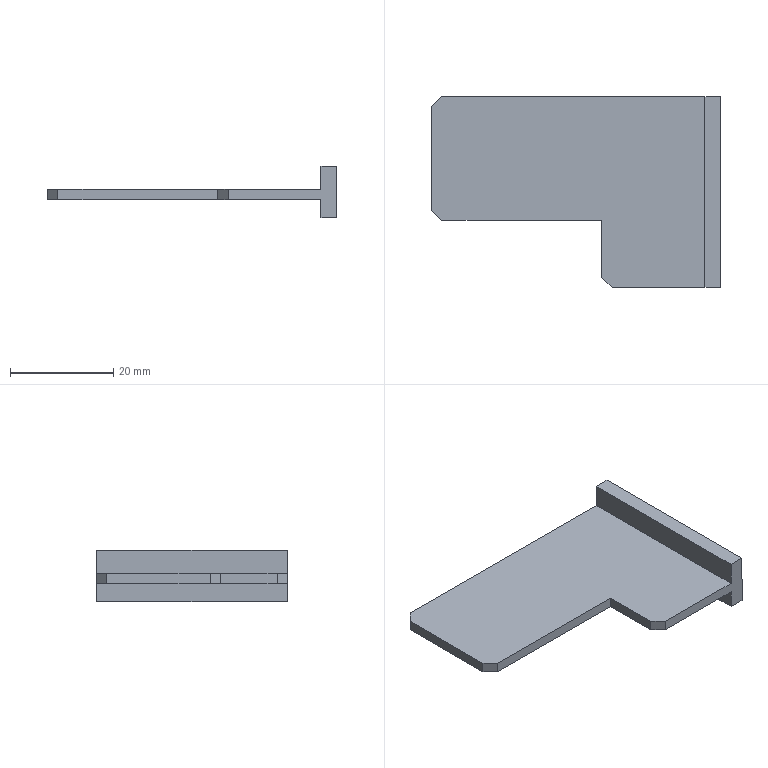Component | SolidWorks | 2023-12-12-28-1 | 1 solid | 15 faces | box 56 x 37 x 10 mm | volume 4162 mm3 | plane 15
build123d program:
from build123d import *

# Parameters (mm, degrees)
SKETCH1_W           = 37
SKETCH1_H           = 56
BOSS_EXTRUDE1_DEPTH = 10
SKETCH2_W           = 4.5
SKETCH2_H           = 53
SKETCH2_W_2         = 3.5
CUT_EXTRUDE1_DEPTH  = 68.86
SKETCH3_W           = 13
SKETCH3_H           = 33
CUT_EXTRUDE2_DEPTH  = 10
CHAMFER1_SIZE       = 2


with BuildPart() as part:
    # Sketch1 → Boss-Extrude1 (new body)
    with BuildSketch(Plane.XY):
        with Locations((18.5, 28)):
            Rectangle(SKETCH1_W, SKETCH1_H)
    extrude(amount=BOSS_EXTRUDE1_DEPTH)

    # Sketch2 → Cut-Extrude1 (cut, through all)
    with BuildSketch(Plane(origin=(37, 0, 0), x_dir=(0, 0, -1), z_dir=(1, 0, 0))):
        with Locations((-7.75, 29.5)):
            Rectangle(SKETCH2_W, SKETCH2_H)
        with Locations((-1.75, 29.5)):
            Rectangle(SKETCH2_W_2, SKETCH2_H)
    extrude(amount=-CUT_EXTRUDE1_DEPTH, mode=Mode.SUBTRACT)

    # Sketch3 → Cut-Extrude2 (cut)
    with BuildSketch(Plane(origin=(0, 0, 3.5), x_dir=(-1, 0, 0), z_dir=(0, 0, -1))):
        with Locations((-6.5, 39.5)):
            Rectangle(SKETCH3_W, SKETCH3_H)
    extrude(amount=-CUT_EXTRUDE2_DEPTH, mode=Mode.SUBTRACT)

    # Chamfer1
    chamfer1_edges = [part.edges().sort_by_distance(p)[0] for p in [
        (37, 56, 4.5),
        (0, 23, 4.5),
        (13, 56, 4.5),
    ]]
    chamfer(chamfer1_edges, length=CHAMFER1_SIZE)


solid = part.part

# Placed as in the assembly
solid = solid.moved(Location((-20.778, -21.367, 78.5), (0, 0, 90)))
STEP:
#1=CARTESIAN_POINT('',(-0.9361,-0.8412,3.307));
#2=VERTEX_POINT('',#1);
#3=CARTESIAN_POINT('',(-1.645,-0.8412,3.307));
#4=VERTEX_POINT('',#3);
#5=CARTESIAN_POINT('',(-0.9361,-0.8412,3.307));
#6=DIRECTION('',(-1.,-0.,-0.));
#7=VECTOR('',#6,39.37);
#8=LINE('',#5,#7);
#9=EDGE_CURVE('',#2,#4,#8,.T.);
#10=ORIENTED_EDGE('',*,*,#9,.T.);
#11=CARTESIAN_POINT('',(-1.645,-0.8412,3.228));
#12=VERTEX_POINT('',#11);
#13=CARTESIAN_POINT('',(-1.645,-0.8412,3.484));
#14=DIRECTION('',(0.,0.,-1.));
#15=VECTOR('',#14,39.37);
#16=LINE('',#13,#15);
#17=EDGE_CURVE('',#4,#12,#16,.T.);
#18=ORIENTED_EDGE('',*,*,#17,.T.);
#19=CARTESIAN_POINT('',(-0.9361,-0.8412,3.228));
#20=VERTEX_POINT('',#19);
#21=CARTESIAN_POINT('',(-3.023,-0.8412,3.228));
#22=DIRECTION('',(1.,0.,0.));
#23=VECTOR('',#22,39.37);
#24=LINE('',#21,#23);
#25=EDGE_CURVE('',#12,#20,#24,.T.);
#26=ORIENTED_EDGE('',*,*,#25,.T.);
#27=CARTESIAN_POINT('',(-0.9361,-0.8412,3.091));
#28=VERTEX_POINT('',#27);
#29=CARTESIAN_POINT('',(-0.9361,-0.8412,3.091));
#30=DIRECTION('',(0.,0.,-1.));
#31=VECTOR('',#30,39.37);
#32=LINE('',#29,#31);
#33=EDGE_CURVE('',#20,#28,#32,.T.);
#34=ORIENTED_EDGE('',*,*,#33,.T.);
#35=CARTESIAN_POINT('',(-0.818,-0.8412,3.091));
#36=VERTEX_POINT('',#35);
#37=CARTESIAN_POINT('',(-0.818,-0.8412,3.091));
#38=DIRECTION('',(1.,0.,0.));
#39=VECTOR('',#38,39.37);
#40=LINE('',#37,#39);
#41=EDGE_CURVE('',#28,#36,#40,.T.);
#42=ORIENTED_EDGE('',*,*,#41,.T.);
#43=CARTESIAN_POINT('',(-0.818,-0.8412,3.484));
#44=VERTEX_POINT('',#43);
#45=CARTESIAN_POINT('',(-0.818,-0.8412,3.484));
#46=DIRECTION('',(0.,0.,-1.));
#47=VECTOR('',#46,39.37);
#48=LINE('',#45,#47);
#49=EDGE_CURVE('',#44,#36,#48,.T.);
#50=ORIENTED_EDGE('',*,*,#49,.F.);
#51=CARTESIAN_POINT('',(-0.9361,-0.8412,3.484));
#52=VERTEX_POINT('',#51);
#53=CARTESIAN_POINT('',(-0.818,-0.8412,3.484));
#54=DIRECTION('',(1.,0.,0.));
#55=VECTOR('',#54,39.37);
#56=LINE('',#53,#55);
#57=EDGE_CURVE('',#52,#44,#56,.T.);
#58=ORIENTED_EDGE('',*,*,#57,.F.);
#59=CARTESIAN_POINT('',(-0.9361,-0.8412,3.484));
#60=DIRECTION('',(0.,0.,-1.));
#61=VECTOR('',#60,39.37);
#62=LINE('',#59,#61);
#63=EDGE_CURVE('',#52,#2,#62,.T.);
#64=ORIENTED_EDGE('',*,*,#63,.T.);
#65=EDGE_LOOP('',(#10,#18,#26,#34,#42,#50,#58,#64));
#66=FACE_OUTER_BOUND('',#65,.T.);
#67=CARTESIAN_POINT('',(-0.818,-0.8412,3.484));
#68=DIRECTION('',(-0.,1.,0.));
#69=DIRECTION('',(0.,0.,-1.));
#70=AXIS2_PLACEMENT_3D('',#67,#68,#69);
#71=PLANE('',#70);
#72=ADVANCED_FACE('',(#66),#71,.F.);
#73=CARTESIAN_POINT('',(-0.818,0.6155,3.091));
#74=VERTEX_POINT('',#73);
#75=CARTESIAN_POINT('',(-0.818,-0.8412,3.091));
#76=DIRECTION('',(-0.,1.,0.));
#77=VECTOR('',#76,39.37);
#78=LINE('',#75,#77);
#79=EDGE_CURVE('',#36,#74,#78,.T.);
#80=ORIENTED_EDGE('',*,*,#79,.T.);
#81=CARTESIAN_POINT('',(-0.818,0.6155,3.484));
#82=VERTEX_POINT('',#81);
#83=CARTESIAN_POINT('',(-0.818,0.6155,3.484));
#84=DIRECTION('',(0.,0.,-1.));
#85=VECTOR('',#84,39.37);
#86=LINE('',#83,#85);
#87=EDGE_CURVE('',#82,#74,#86,.T.);
#88=ORIENTED_EDGE('',*,*,#87,.F.);
#89=CARTESIAN_POINT('',(-0.818,-0.8412,3.484));
#90=DIRECTION('',(-0.,1.,0.));
#91=VECTOR('',#90,39.37);
#92=LINE('',#89,#91);
#93=EDGE_CURVE('',#44,#82,#92,.T.);
#94=ORIENTED_EDGE('',*,*,#93,.F.);
#95=ORIENTED_EDGE('',*,*,#49,.T.);
#96=EDGE_LOOP('',(#80,#88,#94,#95));
#97=FACE_OUTER_BOUND('',#96,.T.);
#98=CARTESIAN_POINT('',(-0.818,-0.8412,3.484));
#99=DIRECTION('',(-1.,-0.,-0.));
#100=DIRECTION('',(-0.,-0.,1.));
#101=AXIS2_PLACEMENT_3D('',#98,#99,#100);
#102=PLANE('',#101);
#103=ADVANCED_FACE('',(#97),#102,.F.);
#104=CARTESIAN_POINT('',(-2.944,0.6155,3.228));
#105=VERTEX_POINT('',#104);
#106=CARTESIAN_POINT('',(-0.9361,0.6155,3.228));
#107=VERTEX_POINT('',#106);
#108=CARTESIAN_POINT('',(-3.023,0.6155,3.228));
#109=DIRECTION('',(1.,0.,0.));
#110=VECTOR('',#109,39.37);
#111=LINE('',#108,#110);
#112=EDGE_CURVE('',#105,#107,#111,.T.);
#113=ORIENTED_EDGE('',*,*,#112,.F.);
#114=CARTESIAN_POINT('',(-2.944,0.6155,3.307));
#115=VERTEX_POINT('',#114);
#116=CARTESIAN_POINT('',(-2.944,0.6155,3.484));
#117=DIRECTION('',(-0.,-0.,1.));
#118=VECTOR('',#117,39.37);
#119=LINE('',#116,#118);
#120=EDGE_CURVE('',#105,#115,#119,.T.);
#121=ORIENTED_EDGE('',*,*,#120,.T.);
#122=CARTESIAN_POINT('',(-0.9361,0.6155,3.307));
#123=VERTEX_POINT('',#122);
#124=CARTESIAN_POINT('',(-0.9361,0.6155,3.307));
#125=DIRECTION('',(-1.,-0.,-0.));
#126=VECTOR('',#125,39.37);
#127=LINE('',#124,#126);
#128=EDGE_CURVE('',#123,#115,#127,.T.);
#129=ORIENTED_EDGE('',*,*,#128,.F.);
#130=CARTESIAN_POINT('',(-0.9361,0.6155,3.484));
#131=VERTEX_POINT('',#130);
#132=CARTESIAN_POINT('',(-0.9361,0.6155,3.484));
#133=DIRECTION('',(0.,0.,-1.));
#134=VECTOR('',#133,39.37);
#135=LINE('',#132,#134);
#136=EDGE_CURVE('',#131,#123,#135,.T.);
#137=ORIENTED_EDGE('',*,*,#136,.F.);
#138=CARTESIAN_POINT('',(-0.818,0.6155,3.484));
#139=DIRECTION('',(-1.,-0.,-0.));
#140=VECTOR('',#139,39.37);
#141=LINE('',#138,#140);
#142=EDGE_CURVE('',#82,#131,#141,.T.);
#143=ORIENTED_EDGE('',*,*,#142,.F.);
#144=ORIENTED_EDGE('',*,*,#87,.T.);
#145=CARTESIAN_POINT('',(-0.9361,0.6155,3.091));
#146=VERTEX_POINT('',#145);
#147=CARTESIAN_POINT('',(-0.818,0.6155,3.091));
#148=DIRECTION('',(-1.,-0.,-0.));
#149=VECTOR('',#148,39.37);
#150=LINE('',#147,#149);
#151=EDGE_CURVE('',#74,#146,#150,.T.);
#152=ORIENTED_EDGE('',*,*,#151,.T.);
#153=CARTESIAN_POINT('',(-0.9361,0.6155,3.091));
#154=DIRECTION('',(0.,0.,-1.));
#155=VECTOR('',#154,39.37);
#156=LINE('',#153,#155);
#157=EDGE_CURVE('',#107,#146,#156,.T.);
#158=ORIENTED_EDGE('',*,*,#157,.F.);
#159=EDGE_LOOP('',(#113,#121,#129,#137,#143,#144,#152,#158));
#160=FACE_OUTER_BOUND('',#159,.T.);
#161=CARTESIAN_POINT('',(-0.818,0.6155,3.484));
#162=DIRECTION('',(0.,-1.,-0.));
#163=DIRECTION('',(-0.,-0.,1.));
#164=AXIS2_PLACEMENT_3D('',#161,#162,#163);
#165=PLANE('',#164);
#166=ADVANCED_FACE('',(#160),#165,.F.);
#167=CARTESIAN_POINT('',(-3.023,-0.2507,3.307));
#168=VERTEX_POINT('',#167);
#169=CARTESIAN_POINT('',(-3.023,0.5367,3.307));
#170=VERTEX_POINT('',#169);
#171=CARTESIAN_POINT('',(-3.023,-0.8412,3.307));
#172=DIRECTION('',(-0.,1.,0.));
#173=VECTOR('',#172,39.37);
#174=LINE('',#171,#173);
#175=EDGE_CURVE('',#168,#170,#174,.T.);
#176=ORIENTED_EDGE('',*,*,#175,.T.);
#177=CARTESIAN_POINT('',(-3.023,0.5367,3.228));
#178=VERTEX_POINT('',#177);
#179=CARTESIAN_POINT('',(-3.023,0.5367,3.484));
#180=DIRECTION('',(0.,0.,-1.));
#181=VECTOR('',#180,39.37);
#182=LINE('',#179,#181);
#183=EDGE_CURVE('',#170,#178,#182,.T.);
#184=ORIENTED_EDGE('',*,*,#183,.T.);
#185=CARTESIAN_POINT('',(-3.023,-0.2507,3.228));
#186=VERTEX_POINT('',#185);
#187=CARTESIAN_POINT('',(-3.023,-0.8412,3.228));
#188=DIRECTION('',(-0.,1.,0.));
#189=VECTOR('',#188,39.37);
#190=LINE('',#187,#189);
#191=EDGE_CURVE('',#186,#178,#190,.T.);
#192=ORIENTED_EDGE('',*,*,#191,.F.);
#193=CARTESIAN_POINT('',(-3.023,-0.2507,3.484));
#194=DIRECTION('',(-0.,-0.,1.));
#195=VECTOR('',#194,39.37);
#196=LINE('',#193,#195);
#197=EDGE_CURVE('',#186,#168,#196,.T.);
#198=ORIENTED_EDGE('',*,*,#197,.T.);
#199=EDGE_LOOP('',(#176,#184,#192,#198));
#200=FACE_OUTER_BOUND('',#199,.T.);
#201=CARTESIAN_POINT('',(-3.023,-0.8412,3.484));
#202=DIRECTION('',(1.,0.,0.));
#203=DIRECTION('',(0.,0.,-1.));
#204=AXIS2_PLACEMENT_3D('',#201,#202,#203);
#205=PLANE('',#204);
#206=ADVANCED_FACE('',(#200),#205,.F.);
#207=ORIENTED_EDGE('',*,*,#142,.T.);
#208=CARTESIAN_POINT('',(-0.9361,-0.8412,3.484));
#209=DIRECTION('',(-0.,1.,0.));
#210=VECTOR('',#209,39.37);
#211=LINE('',#208,#210);
#212=EDGE_CURVE('',#52,#131,#211,.T.);
#213=ORIENTED_EDGE('',*,*,#212,.F.);
#214=ORIENTED_EDGE('',*,*,#57,.T.);
#215=ORIENTED_EDGE('',*,*,#93,.T.);
#216=EDGE_LOOP('',(#207,#213,#214,#215));
#217=FACE_OUTER_BOUND('',#216,.T.);
#218=CARTESIAN_POINT('',(-0.818,-0.8412,3.484));
#219=DIRECTION('',(0.,0.,-1.));
#220=DIRECTION('',(0.,-1.,-0.));
#221=AXIS2_PLACEMENT_3D('',#218,#219,#220);
#222=PLANE('',#221);
#223=ADVANCED_FACE('',(#217),#222,.F.);
#224=CARTESIAN_POINT('',(-0.9361,-0.8412,3.091));
#225=DIRECTION('',(-0.,1.,0.));
#226=VECTOR('',#225,39.37);
#227=LINE('',#224,#226);
#228=EDGE_CURVE('',#28,#146,#227,.T.);
#229=ORIENTED_EDGE('',*,*,#228,.T.);
#230=ORIENTED_EDGE('',*,*,#151,.F.);
#231=ORIENTED_EDGE('',*,*,#79,.F.);
#232=ORIENTED_EDGE('',*,*,#41,.F.);
#233=EDGE_LOOP('',(#229,#230,#231,#232));
#234=FACE_OUTER_BOUND('',#233,.T.);
#235=CARTESIAN_POINT('',(-0.818,-0.8412,3.091));
#236=DIRECTION('',(0.,0.,-1.));
#237=DIRECTION('',(0.,-1.,-0.));
#238=AXIS2_PLACEMENT_3D('',#235,#236,#237);
#239=PLANE('',#238);
#240=ADVANCED_FACE('',(#234),#239,.T.);
#241=ORIENTED_EDGE('',*,*,#157,.T.);
#242=ORIENTED_EDGE('',*,*,#228,.F.);
#243=ORIENTED_EDGE('',*,*,#33,.F.);
#244=CARTESIAN_POINT('',(-0.9361,-0.8412,3.228));
#245=DIRECTION('',(-0.,1.,0.));
#246=VECTOR('',#245,39.37);
#247=LINE('',#244,#246);
#248=EDGE_CURVE('',#20,#107,#247,.T.);
#249=ORIENTED_EDGE('',*,*,#248,.T.);
#250=EDGE_LOOP('',(#241,#242,#243,#249));
#251=FACE_OUTER_BOUND('',#250,.T.);
#252=CARTESIAN_POINT('',(-0.9361,-0.8412,3.091));
#253=DIRECTION('',(1.,0.,0.));
#254=DIRECTION('',(0.,0.,-1.));
#255=AXIS2_PLACEMENT_3D('',#252,#253,#254);
#256=PLANE('',#255);
#257=ADVANCED_FACE('',(#251),#256,.F.);
#258=ORIENTED_EDGE('',*,*,#25,.F.);
#259=CARTESIAN_POINT('',(-1.724,-0.7625,3.228));
#260=VERTEX_POINT('',#259);
#261=CARTESIAN_POINT('',(-1.645,-0.8412,3.228));
#262=DIRECTION('',(-0.7071,0.7071,-0.));
#263=VECTOR('',#262,39.37);
#264=LINE('',#261,#263);
#265=EDGE_CURVE('',#12,#260,#264,.T.);
#266=ORIENTED_EDGE('',*,*,#265,.T.);
#267=CARTESIAN_POINT('',(-1.724,-0.3294,3.228));
#268=VERTEX_POINT('',#267);
#269=CARTESIAN_POINT('',(-1.724,-0.8412,3.228));
#270=DIRECTION('',(0.,-1.,-0.));
#271=VECTOR('',#270,39.37);
#272=LINE('',#269,#271);
#273=EDGE_CURVE('',#268,#260,#272,.T.);
#274=ORIENTED_EDGE('',*,*,#273,.F.);
#275=CARTESIAN_POINT('',(-2.944,-0.3294,3.228));
#276=VERTEX_POINT('',#275);
#277=CARTESIAN_POINT('',(-3.023,-0.3294,3.228));
#278=DIRECTION('',(1.,0.,0.));
#279=VECTOR('',#278,39.37);
#280=LINE('',#277,#279);
#281=EDGE_CURVE('',#276,#268,#280,.T.);
#282=ORIENTED_EDGE('',*,*,#281,.F.);
#283=CARTESIAN_POINT('',(-2.944,-0.3294,3.228));
#284=DIRECTION('',(-0.7071,0.7071,-0.));
#285=VECTOR('',#284,39.37);
#286=LINE('',#283,#285);
#287=EDGE_CURVE('',#276,#186,#286,.T.);
#288=ORIENTED_EDGE('',*,*,#287,.T.);
#289=ORIENTED_EDGE('',*,*,#191,.T.);
#290=CARTESIAN_POINT('',(-3.023,0.5367,3.228));
#291=DIRECTION('',(0.7071,0.7071,0.));
#292=VECTOR('',#291,39.37);
#293=LINE('',#290,#292);
#294=EDGE_CURVE('',#178,#105,#293,.T.);
#295=ORIENTED_EDGE('',*,*,#294,.T.);
#296=ORIENTED_EDGE('',*,*,#112,.T.);
#297=ORIENTED_EDGE('',*,*,#248,.F.);
#298=EDGE_LOOP('',(#258,#266,#274,#282,#288,#289,#295,#296,#297));
#299=FACE_OUTER_BOUND('',#298,.T.);
#300=CARTESIAN_POINT('',(-3.023,-0.8412,3.228));
#301=DIRECTION('',(-0.,-0.,1.));
#302=DIRECTION('',(1.,0.,0.));
#303=AXIS2_PLACEMENT_3D('',#300,#301,#302);
#304=PLANE('',#303);
#305=ADVANCED_FACE('',(#299),#304,.F.);
#306=CARTESIAN_POINT('',(-1.724,-0.3294,3.307));
#307=VERTEX_POINT('',#306);
#308=CARTESIAN_POINT('',(-1.724,-0.7625,3.307));
#309=VERTEX_POINT('',#308);
#310=CARTESIAN_POINT('',(-1.724,-0.8412,3.307));
#311=DIRECTION('',(0.,-1.,-0.));
#312=VECTOR('',#311,39.37);
#313=LINE('',#310,#312);
#314=EDGE_CURVE('',#307,#309,#313,.T.);
#315=ORIENTED_EDGE('',*,*,#314,.T.);
#316=CARTESIAN_POINT('',(-1.645,-0.8412,3.307));
#317=DIRECTION('',(0.7071,-0.7071,0.));
#318=VECTOR('',#317,39.37);
#319=LINE('',#316,#318);
#320=EDGE_CURVE('',#309,#4,#319,.T.);
#321=ORIENTED_EDGE('',*,*,#320,.T.);
#322=ORIENTED_EDGE('',*,*,#9,.F.);
#323=CARTESIAN_POINT('',(-0.9361,-0.8412,3.307));
#324=DIRECTION('',(-0.,1.,0.));
#325=VECTOR('',#324,39.37);
#326=LINE('',#323,#325);
#327=EDGE_CURVE('',#2,#123,#326,.T.);
#328=ORIENTED_EDGE('',*,*,#327,.T.);
#329=ORIENTED_EDGE('',*,*,#128,.T.);
#330=CARTESIAN_POINT('',(-3.023,0.5367,3.307));
#331=DIRECTION('',(-0.7071,-0.7071,-0.));
#332=VECTOR('',#331,39.37);
#333=LINE('',#330,#332);
#334=EDGE_CURVE('',#115,#170,#333,.T.);
#335=ORIENTED_EDGE('',*,*,#334,.T.);
#336=ORIENTED_EDGE('',*,*,#175,.F.);
#337=CARTESIAN_POINT('',(-2.944,-0.3294,3.307));
#338=VERTEX_POINT('',#337);
#339=CARTESIAN_POINT('',(-2.944,-0.3294,3.307));
#340=DIRECTION('',(0.7071,-0.7071,0.));
#341=VECTOR('',#340,39.37);
#342=LINE('',#339,#341);
#343=EDGE_CURVE('',#168,#338,#342,.T.);
#344=ORIENTED_EDGE('',*,*,#343,.T.);
#345=CARTESIAN_POINT('',(-0.9361,-0.3294,3.307));
#346=DIRECTION('',(1.,0.,0.));
#347=VECTOR('',#346,39.37);
#348=LINE('',#345,#347);
#349=EDGE_CURVE('',#338,#307,#348,.T.);
#350=ORIENTED_EDGE('',*,*,#349,.T.);
#351=EDGE_LOOP('',(#315,#321,#322,#328,#329,#335,#336,#344,#350));
#352=FACE_OUTER_BOUND('',#351,.T.);
#353=CARTESIAN_POINT('',(-0.9361,-0.8412,3.307));
#354=DIRECTION('',(0.,0.,-1.));
#355=DIRECTION('',(0.,-1.,-0.));
#356=AXIS2_PLACEMENT_3D('',#353,#354,#355);
#357=PLANE('',#356);
#358=ADVANCED_FACE('',(#352),#357,.F.);
#359=ORIENTED_EDGE('',*,*,#136,.T.);
#360=ORIENTED_EDGE('',*,*,#327,.F.);
#361=ORIENTED_EDGE('',*,*,#63,.F.);
#362=ORIENTED_EDGE('',*,*,#212,.T.);
#363=EDGE_LOOP('',(#359,#360,#361,#362));
#364=FACE_OUTER_BOUND('',#363,.T.);
#365=CARTESIAN_POINT('',(-0.9361,-0.8412,3.484));
#366=DIRECTION('',(1.,0.,0.));
#367=DIRECTION('',(0.,0.,-1.));
#368=AXIS2_PLACEMENT_3D('',#365,#366,#367);
#369=PLANE('',#368);
#370=ADVANCED_FACE('',(#364),#369,.F.);
#371=ORIENTED_EDGE('',*,*,#273,.T.);
#372=CARTESIAN_POINT('',(-1.724,-0.7625,3.622));
#373=DIRECTION('',(-0.,-0.,1.));
#374=VECTOR('',#373,39.37);
#375=LINE('',#372,#374);
#376=EDGE_CURVE('',#260,#309,#375,.T.);
#377=ORIENTED_EDGE('',*,*,#376,.T.);
#378=ORIENTED_EDGE('',*,*,#314,.F.);
#379=CARTESIAN_POINT('',(-1.724,-0.3294,3.622));
#380=DIRECTION('',(0.,0.,-1.));
#381=VECTOR('',#380,39.37);
#382=LINE('',#379,#381);
#383=EDGE_CURVE('',#307,#268,#382,.T.);
#384=ORIENTED_EDGE('',*,*,#383,.T.);
#385=EDGE_LOOP('',(#371,#377,#378,#384));
#386=FACE_OUTER_BOUND('',#385,.T.);
#387=CARTESIAN_POINT('',(-1.724,-0.8412,3.622));
#388=DIRECTION('',(1.,0.,0.));
#389=DIRECTION('',(0.,0.,-1.));
#390=AXIS2_PLACEMENT_3D('',#387,#388,#389);
#391=PLANE('',#390);
#392=ADVANCED_FACE('',(#386),#391,.F.);
#393=ORIENTED_EDGE('',*,*,#349,.F.);
#394=CARTESIAN_POINT('',(-2.944,-0.3294,3.622));
#395=DIRECTION('',(0.,0.,-1.));
#396=VECTOR('',#395,39.37);
#397=LINE('',#394,#396);
#398=EDGE_CURVE('',#338,#276,#397,.T.);
#399=ORIENTED_EDGE('',*,*,#398,.T.);
#400=ORIENTED_EDGE('',*,*,#281,.T.);
#401=ORIENTED_EDGE('',*,*,#383,.F.);
#402=EDGE_LOOP('',(#393,#399,#400,#401));
#403=FACE_OUTER_BOUND('',#402,.T.);
#404=CARTESIAN_POINT('',(-3.023,-0.3294,3.622));
#405=DIRECTION('',(-0.,1.,0.));
#406=DIRECTION('',(-1.,-0.,-0.));
#407=AXIS2_PLACEMENT_3D('',#404,#405,#406);
#408=PLANE('',#407);
#409=ADVANCED_FACE('',(#403),#408,.F.);
#410=ORIENTED_EDGE('',*,*,#320,.F.);
#411=ORIENTED_EDGE('',*,*,#376,.F.);
#412=ORIENTED_EDGE('',*,*,#265,.F.);
#413=ORIENTED_EDGE('',*,*,#17,.F.);
#414=EDGE_LOOP('',(#410,#411,#412,#413));
#415=FACE_OUTER_BOUND('',#414,.T.);
#416=CARTESIAN_POINT('',(-1.645,-0.8412,3.484));
#417=DIRECTION('',(0.7071,0.7071,0.));
#418=DIRECTION('',(0.,0.,-1.));
#419=AXIS2_PLACEMENT_3D('',#416,#417,#418);
#420=PLANE('',#419);
#421=ADVANCED_FACE('',(#415),#420,.F.);
#422=ORIENTED_EDGE('',*,*,#334,.F.);
#423=ORIENTED_EDGE('',*,*,#120,.F.);
#424=ORIENTED_EDGE('',*,*,#294,.F.);
#425=ORIENTED_EDGE('',*,*,#183,.F.);
#426=EDGE_LOOP('',(#422,#423,#424,#425));
#427=FACE_OUTER_BOUND('',#426,.T.);
#428=CARTESIAN_POINT('',(-3.023,0.5367,3.484));
#429=DIRECTION('',(0.7071,-0.7071,0.));
#430=DIRECTION('',(0.,0.,-1.));
#431=AXIS2_PLACEMENT_3D('',#428,#429,#430);
#432=PLANE('',#431);
#433=ADVANCED_FACE('',(#427),#432,.F.);
#434=ORIENTED_EDGE('',*,*,#343,.F.);
#435=ORIENTED_EDGE('',*,*,#197,.F.);
#436=ORIENTED_EDGE('',*,*,#287,.F.);
#437=ORIENTED_EDGE('',*,*,#398,.F.);
#438=EDGE_LOOP('',(#434,#435,#436,#437));
#439=FACE_OUTER_BOUND('',#438,.T.);
#440=CARTESIAN_POINT('',(-2.944,-0.3294,3.622));
#441=DIRECTION('',(0.7071,0.7071,0.));
#442=DIRECTION('',(0.,0.,-1.));
#443=AXIS2_PLACEMENT_3D('',#440,#441,#442);
#444=PLANE('',#443);
#445=ADVANCED_FACE('',(#439),#444,.F.);
#446=CLOSED_SHELL('',(#72,#103,#166,#206,#223,#240,#257,#305,#358,#370,#392,#409,#421,#433,#445));
#447=MANIFOLD_SOLID_BREP('',#446);
#448=CARTESIAN_POINT('',(0.,0.,0.));
#449=DIRECTION('',(0.,0.,1.));
#450=DIRECTION('',(1.,0.,0.));
#451=AXIS2_PLACEMENT_3D('',#448,#449,#450);
#452=(LENGTH_UNIT()NAMED_UNIT(*)SI_UNIT($,.METRE.));
#453=LENGTH_MEASURE_WITH_UNIT(LENGTH_MEASURE(0.0254),#452);
#454=DIMENSIONAL_EXPONENTS(1.,0.,0.,0.,0.,0.,0.);
#455=(CONVERSION_BASED_UNIT('',#453)LENGTH_UNIT()NAMED_UNIT(#454));
#456=UNCERTAINTY_MEASURE_WITH_UNIT(LENGTH_MEASURE(0.00001),#455,'','');
#457=(NAMED_UNIT(*)PLANE_ANGLE_UNIT()SI_UNIT($,.RADIAN.));
#458=(NAMED_UNIT(*)SI_UNIT($,.STERADIAN.)SOLID_ANGLE_UNIT());
#459=(GEOMETRIC_REPRESENTATION_CONTEXT(3)GLOBAL_UNCERTAINTY_ASSIGNED_CONTEXT((#456))GLOBAL_UNIT_ASSIGNED_CONTEXT((#455,#457,#458))REPRESENTATION_CONTEXT('',''));
#460=ADVANCED_BREP_SHAPE_REPRESENTATION('',(#447,#451),#459);
#461=COLOUR_RGB('',0.7922,0.8196,0.9333);
#462=FILL_AREA_STYLE_COLOUR('',#461);
#463=FILL_AREA_STYLE('',(#462));
#464=SURFACE_STYLE_FILL_AREA(#463);
#465=SURFACE_SIDE_STYLE('',(#464));
#466=SURFACE_STYLE_USAGE(.BOTH.,#465);
#467=PRESENTATION_STYLE_ASSIGNMENT((#466));
#468=STYLED_ITEM('',(#467),#447);
#469=PRESENTATION_LAYER_ASSIGNMENT('','',(#468));
#470=(LENGTH_UNIT()NAMED_UNIT(*)SI_UNIT($,.METRE.));
#471=LENGTH_MEASURE_WITH_UNIT(LENGTH_MEASURE(0.0254),#470);
#472=DIMENSIONAL_EXPONENTS(1.,0.,0.,0.,0.,0.,0.);
#473=(CONVERSION_BASED_UNIT('',#471)LENGTH_UNIT()NAMED_UNIT(#472));
#474=UNCERTAINTY_MEASURE_WITH_UNIT(LENGTH_MEASURE(0.00001),#473,'','');
#475=(NAMED_UNIT(*)PLANE_ANGLE_UNIT()SI_UNIT($,.RADIAN.));
#476=(NAMED_UNIT(*)SI_UNIT($,.STERADIAN.)SOLID_ANGLE_UNIT());
#477=(GEOMETRIC_REPRESENTATION_CONTEXT(3)GLOBAL_UNCERTAINTY_ASSIGNED_CONTEXT((#474))GLOBAL_UNIT_ASSIGNED_CONTEXT((#473,#475,#476))REPRESENTATION_CONTEXT('',''));
#478=MECHANICAL_DESIGN_GEOMETRIC_PRESENTATION_REPRESENTATION('',(#468),#477);